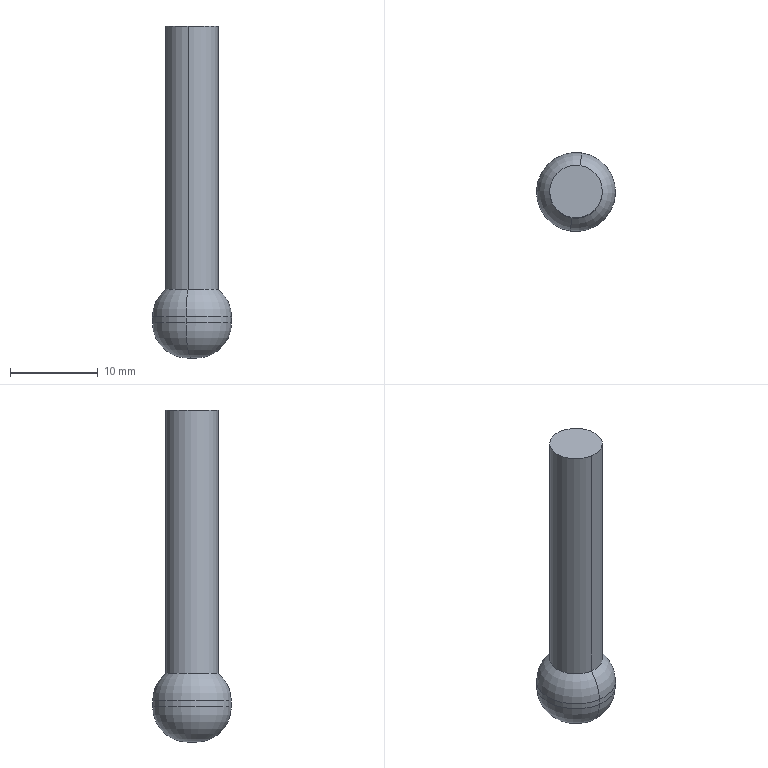Component | SolidWorks | 03-MillingCutterHead-1 | 1 solid | 10 faces | box 9 x 9 x 37.8 mm | volume 1230 mm3 | torus 4 | cylinder 4 | plane 2 | commonest cylinder face diameters 9 x2 6 x2
STEP:
#1=COLOUR_RGB('',0.7922,0.8196,0.9333);
#2=FILL_AREA_STYLE_COLOUR('',#1);
#3=FILL_AREA_STYLE('',(#2));
#4=SURFACE_STYLE_FILL_AREA(#3);
#5=SURFACE_SIDE_STYLE('',(#4));
#6=SURFACE_STYLE_USAGE(.BOTH.,#5);
#7=PRESENTATION_STYLE_ASSIGNMENT((#6));
#8=CARTESIAN_POINT('',(-1.942,3.463,-8.391));
#9=VERTEX_POINT('',#8);
#10=CARTESIAN_POINT('',(-1.995,3.112,-8.391));
#11=VERTEX_POINT('',#10);
#12=CARTESIAN_POINT('',(-1.969,3.287,-8.391));
#13=DIRECTION('',(0.,-0.,-1.));
#14=DIRECTION('',(-0.1517,-0.9884,0.));
#15=AXIS2_PLACEMENT_3D('',#12,#13,#14);
#16=CIRCLE('',#15,0.1772);
#17=EDGE_CURVE('',#9,#11,#16,.T.);
#18=ORIENTED_EDGE('',*,*,#17,.F.);
#19=CARTESIAN_POINT('',(-1.951,3.404,-8.268));
#20=VERTEX_POINT('',#19);
#21=CARTESIAN_POINT('',(-1.966,3.307,-8.391));
#22=DIRECTION('',(0.9884,-0.1517,0.));
#23=DIRECTION('',(0.1517,0.9884,0.));
#24=AXIS2_PLACEMENT_3D('',#21,#22,#23);
#25=CIRCLE('',#24,0.1575);
#26=EDGE_CURVE('',#9,#20,#25,.T.);
#27=ORIENTED_EDGE('',*,*,#26,.T.);
#28=CARTESIAN_POINT('',(-1.986,3.171,-8.268));
#29=VERTEX_POINT('',#28);
#30=CARTESIAN_POINT('',(-1.969,3.287,-8.268));
#31=DIRECTION('',(0.,-0.,-1.));
#32=DIRECTION('',(0.1517,0.9884,0.));
#33=AXIS2_PLACEMENT_3D('',#30,#31,#32);
#34=CIRCLE('',#33,0.1181);
#35=EDGE_CURVE('',#20,#29,#34,.T.);
#36=ORIENTED_EDGE('',*,*,#35,.T.);
#37=CARTESIAN_POINT('',(-1.971,3.268,-8.391));
#38=DIRECTION('',(-0.9884,0.1517,-0.));
#39=DIRECTION('',(-0.1517,-0.9884,0.));
#40=AXIS2_PLACEMENT_3D('',#37,#38,#39);
#41=CIRCLE('',#40,0.1575);
#42=EDGE_CURVE('',#11,#29,#41,.T.);
#43=ORIENTED_EDGE('',*,*,#42,.F.);
#44=EDGE_LOOP('',(#18,#27,#36,#43));
#45=FACE_OUTER_BOUND('',#44,.T.);
#46=CARTESIAN_POINT('',(-1.969,3.287,-8.391));
#47=DIRECTION('',(-0.,0.,1.));
#48=DIRECTION('',(-0.1517,-0.9884,0.));
#49=AXIS2_PLACEMENT_3D('',#46,#47,#48);
#50=TOROIDAL_SURFACE('',#49,0.01969,0.1575);
#51=ADVANCED_FACE('',(#45),#50,.T.);
#52=CARTESIAN_POINT('',(-1.995,3.112,-8.417));
#53=VERTEX_POINT('',#52);
#54=CARTESIAN_POINT('',(-1.942,3.463,-8.417));
#55=VERTEX_POINT('',#54);
#56=CARTESIAN_POINT('',(-1.969,3.287,-8.417));
#57=DIRECTION('',(-0.,0.,1.));
#58=DIRECTION('',(0.1517,0.9884,0.));
#59=AXIS2_PLACEMENT_3D('',#56,#57,#58);
#60=CIRCLE('',#59,0.1772);
#61=EDGE_CURVE('',#53,#55,#60,.T.);
#62=ORIENTED_EDGE('',*,*,#61,.F.);
#63=CARTESIAN_POINT('',(-1.971,3.268,-8.575));
#64=VERTEX_POINT('',#63);
#65=CARTESIAN_POINT('',(-1.971,3.268,-8.417));
#66=DIRECTION('',(0.9884,-0.1517,0.));
#67=DIRECTION('',(0.1517,0.9884,0.));
#68=AXIS2_PLACEMENT_3D('',#65,#66,#67);
#69=CIRCLE('',#68,0.1575);
#70=EDGE_CURVE('',#53,#64,#69,.T.);
#71=ORIENTED_EDGE('',*,*,#70,.T.);
#72=CARTESIAN_POINT('',(-1.966,3.307,-8.575));
#73=VERTEX_POINT('',#72);
#74=CARTESIAN_POINT('',(-1.969,3.287,-8.575));
#75=DIRECTION('',(0.,-0.,-1.));
#76=DIRECTION('',(0.1517,0.9884,0.));
#77=AXIS2_PLACEMENT_3D('',#74,#75,#76);
#78=CIRCLE('',#77,0.01969);
#79=EDGE_CURVE('',#73,#64,#78,.T.);
#80=ORIENTED_EDGE('',*,*,#79,.F.);
#81=CARTESIAN_POINT('',(-1.966,3.307,-8.417));
#82=DIRECTION('',(-0.9884,0.1517,-0.));
#83=DIRECTION('',(-0.1517,-0.9884,0.));
#84=AXIS2_PLACEMENT_3D('',#81,#82,#83);
#85=CIRCLE('',#84,0.1575);
#86=EDGE_CURVE('',#55,#73,#85,.T.);
#87=ORIENTED_EDGE('',*,*,#86,.F.);
#88=EDGE_LOOP('',(#62,#71,#80,#87));
#89=FACE_OUTER_BOUND('',#88,.T.);
#90=CARTESIAN_POINT('',(-1.969,3.287,-8.417));
#91=DIRECTION('',(0.,-0.,-1.));
#92=DIRECTION('',(0.1517,0.9884,-0.));
#93=AXIS2_PLACEMENT_3D('',#90,#91,#92);
#94=TOROIDAL_SURFACE('',#93,0.01969,0.1575);
#95=ADVANCED_FACE('',(#89),#94,.T.);
#96=ORIENTED_EDGE('',*,*,#61,.T.);
#97=CARTESIAN_POINT('',(-1.942,3.463,-8.575));
#98=DIRECTION('',(-0.,0.,1.));
#99=VECTOR('',#98,39.37);
#100=LINE('',#97,#99);
#101=EDGE_CURVE('',#55,#9,#100,.T.);
#102=ORIENTED_EDGE('',*,*,#101,.T.);
#103=ORIENTED_EDGE('',*,*,#17,.T.);
#104=CARTESIAN_POINT('',(-1.995,3.112,-8.575));
#105=DIRECTION('',(-0.,0.,1.));
#106=VECTOR('',#105,39.37);
#107=LINE('',#104,#106);
#108=EDGE_CURVE('',#53,#11,#107,.T.);
#109=ORIENTED_EDGE('',*,*,#108,.F.);
#110=EDGE_LOOP('',(#96,#102,#103,#109));
#111=FACE_OUTER_BOUND('',#110,.T.);
#112=CARTESIAN_POINT('',(-1.969,3.287,-8.575));
#113=DIRECTION('',(-0.,0.,1.));
#114=DIRECTION('',(-0.1517,-0.9884,0.));
#115=AXIS2_PLACEMENT_3D('',#112,#113,#114);
#116=CYLINDRICAL_SURFACE('',#115,0.1772);
#117=ADVANCED_FACE('',(#111),#116,.T.);
#118=ORIENTED_EDGE('',*,*,#35,.F.);
#119=CARTESIAN_POINT('',(-1.951,3.404,-7.087));
#120=VERTEX_POINT('',#119);
#121=CARTESIAN_POINT('',(-1.951,3.404,-8.268));
#122=DIRECTION('',(-0.,0.,1.));
#123=VECTOR('',#122,39.37);
#124=LINE('',#121,#123);
#125=EDGE_CURVE('',#20,#120,#124,.T.);
#126=ORIENTED_EDGE('',*,*,#125,.T.);
#127=CARTESIAN_POINT('',(-1.986,3.171,-7.087));
#128=VERTEX_POINT('',#127);
#129=CARTESIAN_POINT('',(-1.969,3.287,-7.087));
#130=DIRECTION('',(-0.,0.,1.));
#131=DIRECTION('',(-0.1517,-0.9884,0.));
#132=AXIS2_PLACEMENT_3D('',#129,#130,#131);
#133=CIRCLE('',#132,0.1181);
#134=EDGE_CURVE('',#128,#120,#133,.T.);
#135=ORIENTED_EDGE('',*,*,#134,.F.);
#136=CARTESIAN_POINT('',(-1.986,3.171,-8.268));
#137=DIRECTION('',(-0.,0.,1.));
#138=VECTOR('',#137,39.37);
#139=LINE('',#136,#138);
#140=EDGE_CURVE('',#29,#128,#139,.T.);
#141=ORIENTED_EDGE('',*,*,#140,.F.);
#142=EDGE_LOOP('',(#118,#126,#135,#141));
#143=FACE_OUTER_BOUND('',#142,.T.);
#144=CARTESIAN_POINT('',(-1.969,3.287,-8.268));
#145=DIRECTION('',(-0.,0.,1.));
#146=DIRECTION('',(-0.1517,-0.9884,0.));
#147=AXIS2_PLACEMENT_3D('',#144,#145,#146);
#148=CYLINDRICAL_SURFACE('',#147,0.1181);
#149=ADVANCED_FACE('',(#143),#148,.T.);
#150=ORIENTED_EDGE('',*,*,#125,.F.);
#151=CARTESIAN_POINT('',(-1.969,3.287,-8.268));
#152=DIRECTION('',(0.,-0.,-1.));
#153=DIRECTION('',(0.1517,0.9884,0.));
#154=AXIS2_PLACEMENT_3D('',#151,#152,#153);
#155=CIRCLE('',#154,0.1181);
#156=EDGE_CURVE('',#29,#20,#155,.T.);
#157=ORIENTED_EDGE('',*,*,#156,.F.);
#158=ORIENTED_EDGE('',*,*,#140,.T.);
#159=CARTESIAN_POINT('',(-1.969,3.287,-7.087));
#160=DIRECTION('',(-0.,0.,1.));
#161=DIRECTION('',(-0.1517,-0.9884,0.));
#162=AXIS2_PLACEMENT_3D('',#159,#160,#161);
#163=CIRCLE('',#162,0.1181);
#164=EDGE_CURVE('',#120,#128,#163,.T.);
#165=ORIENTED_EDGE('',*,*,#164,.F.);
#166=EDGE_LOOP('',(#150,#157,#158,#165));
#167=FACE_OUTER_BOUND('',#166,.T.);
#168=CARTESIAN_POINT('',(-1.969,3.287,-8.268));
#169=DIRECTION('',(-0.,0.,1.));
#170=DIRECTION('',(-0.1517,-0.9884,0.));
#171=AXIS2_PLACEMENT_3D('',#168,#169,#170);
#172=CYLINDRICAL_SURFACE('',#171,0.1181);
#173=ADVANCED_FACE('',(#167),#172,.T.);
#174=ORIENTED_EDGE('',*,*,#101,.F.);
#175=CARTESIAN_POINT('',(-1.969,3.287,-8.417));
#176=DIRECTION('',(-0.,0.,1.));
#177=DIRECTION('',(0.1517,0.9884,0.));
#178=AXIS2_PLACEMENT_3D('',#175,#176,#177);
#179=CIRCLE('',#178,0.1772);
#180=EDGE_CURVE('',#55,#53,#179,.T.);
#181=ORIENTED_EDGE('',*,*,#180,.T.);
#182=ORIENTED_EDGE('',*,*,#108,.T.);
#183=CARTESIAN_POINT('',(-1.969,3.287,-8.391));
#184=DIRECTION('',(0.,-0.,-1.));
#185=DIRECTION('',(-0.1517,-0.9884,0.));
#186=AXIS2_PLACEMENT_3D('',#183,#184,#185);
#187=CIRCLE('',#186,0.1772);
#188=EDGE_CURVE('',#11,#9,#187,.T.);
#189=ORIENTED_EDGE('',*,*,#188,.T.);
#190=EDGE_LOOP('',(#174,#181,#182,#189));
#191=FACE_OUTER_BOUND('',#190,.T.);
#192=CARTESIAN_POINT('',(-1.969,3.287,-8.575));
#193=DIRECTION('',(-0.,0.,1.));
#194=DIRECTION('',(-0.1517,-0.9884,0.));
#195=AXIS2_PLACEMENT_3D('',#192,#193,#194);
#196=CYLINDRICAL_SURFACE('',#195,0.1772);
#197=ADVANCED_FACE('',(#191),#196,.T.);
#198=ORIENTED_EDGE('',*,*,#79,.T.);
#199=CARTESIAN_POINT('',(-1.969,3.287,-8.575));
#200=DIRECTION('',(0.,-0.,-1.));
#201=DIRECTION('',(0.1517,0.9884,0.));
#202=AXIS2_PLACEMENT_3D('',#199,#200,#201);
#203=CIRCLE('',#202,0.01969);
#204=EDGE_CURVE('',#64,#73,#203,.T.);
#205=ORIENTED_EDGE('',*,*,#204,.T.);
#206=EDGE_LOOP('',(#198,#205));
#207=FACE_OUTER_BOUND('',#206,.T.);
#208=CARTESIAN_POINT('',(-1.969,3.287,-8.575));
#209=DIRECTION('',(0.,-0.,-1.));
#210=DIRECTION('',(0.1517,0.9884,-0.));
#211=AXIS2_PLACEMENT_3D('',#208,#209,#210);
#212=PLANE('',#211);
#213=ADVANCED_FACE('',(#207),#212,.T.);
#214=ORIENTED_EDGE('',*,*,#70,.F.);
#215=ORIENTED_EDGE('',*,*,#180,.F.);
#216=ORIENTED_EDGE('',*,*,#86,.T.);
#217=ORIENTED_EDGE('',*,*,#204,.F.);
#218=EDGE_LOOP('',(#214,#215,#216,#217));
#219=FACE_OUTER_BOUND('',#218,.T.);
#220=CARTESIAN_POINT('',(-1.969,3.287,-8.417));
#221=DIRECTION('',(0.,-0.,-1.));
#222=DIRECTION('',(0.1517,0.9884,-0.));
#223=AXIS2_PLACEMENT_3D('',#220,#221,#222);
#224=TOROIDAL_SURFACE('',#223,0.01969,0.1575);
#225=ADVANCED_FACE('',(#219),#224,.T.);
#226=ORIENTED_EDGE('',*,*,#26,.F.);
#227=ORIENTED_EDGE('',*,*,#188,.F.);
#228=ORIENTED_EDGE('',*,*,#42,.T.);
#229=ORIENTED_EDGE('',*,*,#156,.T.);
#230=EDGE_LOOP('',(#226,#227,#228,#229));
#231=FACE_OUTER_BOUND('',#230,.T.);
#232=CARTESIAN_POINT('',(-1.969,3.287,-8.391));
#233=DIRECTION('',(-0.,0.,1.));
#234=DIRECTION('',(-0.1517,-0.9884,0.));
#235=AXIS2_PLACEMENT_3D('',#232,#233,#234);
#236=TOROIDAL_SURFACE('',#235,0.01969,0.1575);
#237=ADVANCED_FACE('',(#231),#236,.T.);
#238=ORIENTED_EDGE('',*,*,#134,.T.);
#239=ORIENTED_EDGE('',*,*,#164,.T.);
#240=EDGE_LOOP('',(#238,#239));
#241=FACE_OUTER_BOUND('',#240,.T.);
#242=CARTESIAN_POINT('',(-1.467,3.962,-7.087));
#243=DIRECTION('',(-0.,0.,1.));
#244=DIRECTION('',(-0.1517,-0.9884,0.));
#245=AXIS2_PLACEMENT_3D('',#242,#243,#244);
#246=PLANE('',#245);
#247=ADVANCED_FACE('',(#241),#246,.T.);
#248=CLOSED_SHELL('',(#51,#95,#117,#149,#173,#197,#213,#225,#237,#247));
#249=MANIFOLD_SOLID_BREP('',#248);
#250=STYLED_ITEM('',(#7),#249);
#251=PRESENTATION_LAYER_ASSIGNMENT('','',(#250));
#252=CARTESIAN_POINT('',(0.,0.,0.));
#253=DIRECTION('',(0.,0.,1.));
#254=DIRECTION('',(1.,0.,0.));
#255=AXIS2_PLACEMENT_3D('',#252,#253,#254);
#256=(LENGTH_UNIT()NAMED_UNIT(*)SI_UNIT($,.METRE.));
#257=LENGTH_MEASURE_WITH_UNIT(LENGTH_MEASURE(0.0254),#256);
#258=DIMENSIONAL_EXPONENTS(1.,0.,0.,0.,0.,0.,0.);
#259=(CONVERSION_BASED_UNIT('',#257)LENGTH_UNIT()NAMED_UNIT(#258));
#260=UNCERTAINTY_MEASURE_WITH_UNIT(LENGTH_MEASURE(0.00001),#259,'','');
#261=(NAMED_UNIT(*)PLANE_ANGLE_UNIT()SI_UNIT($,.RADIAN.));
#262=(NAMED_UNIT(*)SI_UNIT($,.STERADIAN.)SOLID_ANGLE_UNIT());
#263=(GEOMETRIC_REPRESENTATION_CONTEXT(3)GLOBAL_UNCERTAINTY_ASSIGNED_CONTEXT((#260))GLOBAL_UNIT_ASSIGNED_CONTEXT((#259,#261,#262))REPRESENTATION_CONTEXT('',''));
#264=ADVANCED_BREP_SHAPE_REPRESENTATION('',(#249,#255),#263);
#265=(LENGTH_UNIT()NAMED_UNIT(*)SI_UNIT($,.METRE.));
#266=LENGTH_MEASURE_WITH_UNIT(LENGTH_MEASURE(0.0254),#265);
#267=DIMENSIONAL_EXPONENTS(1.,0.,0.,0.,0.,0.,0.);
#268=(CONVERSION_BASED_UNIT('',#266)LENGTH_UNIT()NAMED_UNIT(#267));
#269=UNCERTAINTY_MEASURE_WITH_UNIT(LENGTH_MEASURE(0.00001),#268,'','');
#270=(NAMED_UNIT(*)PLANE_ANGLE_UNIT()SI_UNIT($,.RADIAN.));
#271=(NAMED_UNIT(*)SI_UNIT($,.STERADIAN.)SOLID_ANGLE_UNIT());
#272=(GEOMETRIC_REPRESENTATION_CONTEXT(3)GLOBAL_UNCERTAINTY_ASSIGNED_CONTEXT((#269))GLOBAL_UNIT_ASSIGNED_CONTEXT((#268,#270,#271))REPRESENTATION_CONTEXT('',''));
#273=MECHANICAL_DESIGN_GEOMETRIC_PRESENTATION_REPRESENTATION('',(#250),#272);